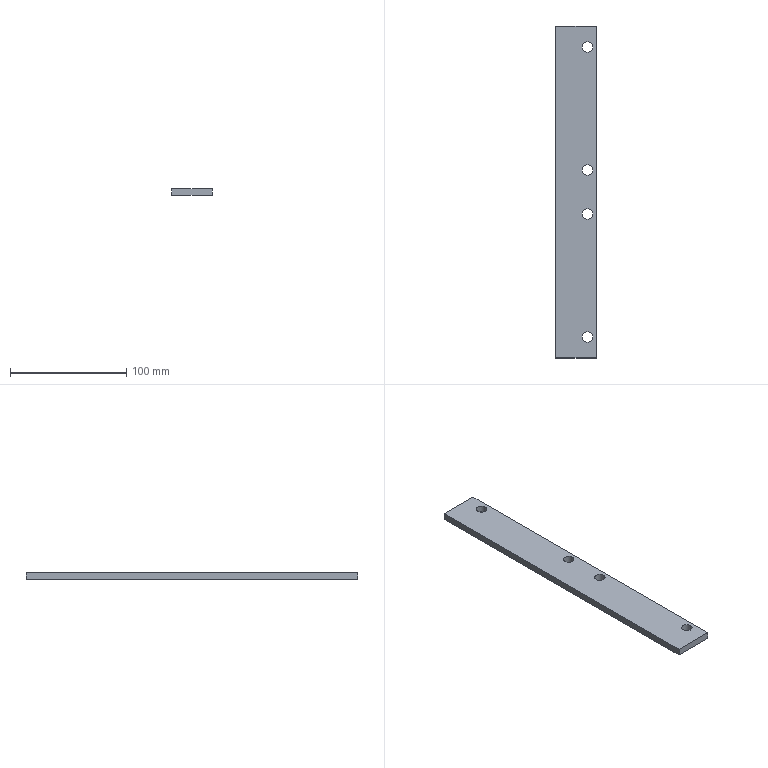Component | NX | FIXED_PLATE_8 | 1 solid | 10 faces | box 35 x 286 x 6 mm | volume 58533 mm3 | plane 6 | cylinder 4 | commonest cylinder face diameters 9 x4
STEP:
#1=CARTESIAN_POINT('',(0.,0.,0.));
#2=DIRECTION('',(0.,0.,1.));
#3=DIRECTION('',(1.,0.,0.));
#4=AXIS2_PLACEMENT_3D('',#1,#2,#3);
#5=CARTESIAN_POINT('',(1499.254,1431.,809.574));
#6=VERTEX_POINT('',#5);
#7=CARTESIAN_POINT('',(1499.254,1145.,809.574));
#8=VERTEX_POINT('',#7);
#9=CARTESIAN_POINT('',(1499.254,1431.,809.574));
#10=DIRECTION('',(-0.,-1.,0.));
#11=VECTOR('',#10,1.);
#12=LINE('',#9,#11);
#13=CARTESIAN_POINT('',(1499.254,1431.,803.574));
#14=DIRECTION('',(-1.,0.,0.));
#15=DIRECTION('',(-0.,-1.,0.));
#16=AXIS2_PLACEMENT_3D('',#13,#14,#15);
#17=PLANE('',#16);
#18=CARTESIAN_POINT('',(0.,6.));
#19=DIRECTION('',(1.,0.));
#20=VECTOR('',#19,1.);
#21=LINE('',#18,#20);
#22=(GEOMETRIC_REPRESENTATION_CONTEXT(2)PARAMETRIC_REPRESENTATION_CONTEXT()REPRESENTATION_CONTEXT('',''));
#23=DEFINITIONAL_REPRESENTATION('',(#21),#22);
#24=PCURVE('',#17,#23);
#25=CARTESIAN_POINT('',(1526.754,1163.,809.574));
#26=DIRECTION('',(0.,0.,1.));
#27=DIRECTION('',(1.,0.,0.));
#28=AXIS2_PLACEMENT_3D('',#25,#26,#27);
#29=PLANE('',#28);
#30=CARTESIAN_POINT('',(-27.5,268.));
#31=DIRECTION('',(-0.,-1.));
#32=VECTOR('',#31,1.);
#33=LINE('',#30,#32);
#34=(GEOMETRIC_REPRESENTATION_CONTEXT(2)PARAMETRIC_REPRESENTATION_CONTEXT()REPRESENTATION_CONTEXT('',''));
#35=DEFINITIONAL_REPRESENTATION('',(#33),#34);
#36=PCURVE('',#29,#35);
#37=SURFACE_CURVE('',#12,(#24,#36),.PCURVE_S1.);
#38=EDGE_CURVE('',#6,#8,#37,.T.);
#39=ORIENTED_EDGE('',*,*,#38,.F.);
#40=CARTESIAN_POINT('',(1499.254,1431.,803.574));
#41=VERTEX_POINT('',#40);
#42=CARTESIAN_POINT('',(1499.254,1431.,803.574));
#43=DIRECTION('',(0.,0.,1.));
#44=VECTOR('',#43,1.);
#45=LINE('',#42,#44);
#46=CARTESIAN_POINT('',(0.,0.));
#47=DIRECTION('',(0.,1.));
#48=VECTOR('',#47,1.);
#49=LINE('',#46,#48);
#50=(GEOMETRIC_REPRESENTATION_CONTEXT(2)PARAMETRIC_REPRESENTATION_CONTEXT()REPRESENTATION_CONTEXT('',''));
#51=DEFINITIONAL_REPRESENTATION('',(#49),#50);
#52=PCURVE('',#17,#51);
#53=CARTESIAN_POINT('',(1534.254,1431.,803.574));
#54=DIRECTION('',(0.,1.,0.));
#55=DIRECTION('',(0.,0.,1.));
#56=AXIS2_PLACEMENT_3D('',#53,#54,#55);
#57=PLANE('',#56);
#58=CARTESIAN_POINT('',(0.,-35.));
#59=DIRECTION('',(1.,0.));
#60=VECTOR('',#59,1.);
#61=LINE('',#58,#60);
#62=(GEOMETRIC_REPRESENTATION_CONTEXT(2)PARAMETRIC_REPRESENTATION_CONTEXT()REPRESENTATION_CONTEXT('',''));
#63=DEFINITIONAL_REPRESENTATION('',(#61),#62);
#64=PCURVE('',#57,#63);
#65=SURFACE_CURVE('',#45,(#52,#64),.PCURVE_S1.);
#66=EDGE_CURVE('',#41,#6,#65,.T.);
#67=ORIENTED_EDGE('',*,*,#66,.F.);
#68=CARTESIAN_POINT('',(1499.254,1145.,803.574));
#69=VERTEX_POINT('',#68);
#70=CARTESIAN_POINT('',(1499.254,1431.,803.574));
#71=DIRECTION('',(-0.,-1.,0.));
#72=VECTOR('',#71,1.);
#73=LINE('',#70,#72);
#74=CARTESIAN_POINT('',(0.,0.));
#75=DIRECTION('',(1.,0.));
#76=VECTOR('',#75,1.);
#77=LINE('',#74,#76);
#78=(GEOMETRIC_REPRESENTATION_CONTEXT(2)PARAMETRIC_REPRESENTATION_CONTEXT()REPRESENTATION_CONTEXT('',''));
#79=DEFINITIONAL_REPRESENTATION('',(#77),#78);
#80=PCURVE('',#17,#79);
#81=CARTESIAN_POINT('',(1526.754,1163.,803.574));
#82=DIRECTION('',(0.,0.,1.));
#83=DIRECTION('',(1.,0.,0.));
#84=AXIS2_PLACEMENT_3D('',#81,#82,#83);
#85=PLANE('',#84);
#86=CARTESIAN_POINT('',(-27.5,268.));
#87=DIRECTION('',(-0.,-1.));
#88=VECTOR('',#87,1.);
#89=LINE('',#86,#88);
#90=(GEOMETRIC_REPRESENTATION_CONTEXT(2)PARAMETRIC_REPRESENTATION_CONTEXT()REPRESENTATION_CONTEXT('',''));
#91=DEFINITIONAL_REPRESENTATION('',(#89),#90);
#92=PCURVE('',#85,#91);
#93=SURFACE_CURVE('',#73,(#80,#92),.PCURVE_S1.);
#94=EDGE_CURVE('',#41,#69,#93,.T.);
#95=ORIENTED_EDGE('',*,*,#94,.T.);
#96=CARTESIAN_POINT('',(1499.254,1145.,803.574));
#97=DIRECTION('',(0.,0.,1.));
#98=VECTOR('',#97,1.);
#99=LINE('',#96,#98);
#100=CARTESIAN_POINT('',(286.,0.));
#101=DIRECTION('',(0.,1.));
#102=VECTOR('',#101,1.);
#103=LINE('',#100,#102);
#104=(GEOMETRIC_REPRESENTATION_CONTEXT(2)PARAMETRIC_REPRESENTATION_CONTEXT()REPRESENTATION_CONTEXT('',''));
#105=DEFINITIONAL_REPRESENTATION('',(#103),#104);
#106=PCURVE('',#17,#105);
#107=CARTESIAN_POINT('',(1499.254,1145.,803.574));
#108=DIRECTION('',(0.,-1.,0.));
#109=DIRECTION('',(0.,0.,-1.));
#110=AXIS2_PLACEMENT_3D('',#107,#108,#109);
#111=PLANE('',#110);
#112=CARTESIAN_POINT('',(0.,0.));
#113=DIRECTION('',(-1.,0.));
#114=VECTOR('',#113,1.);
#115=LINE('',#112,#114);
#116=(GEOMETRIC_REPRESENTATION_CONTEXT(2)PARAMETRIC_REPRESENTATION_CONTEXT()REPRESENTATION_CONTEXT('',''));
#117=DEFINITIONAL_REPRESENTATION('',(#115),#116);
#118=PCURVE('',#111,#117);
#119=SURFACE_CURVE('',#99,(#106,#118),.PCURVE_S1.);
#120=EDGE_CURVE('',#69,#8,#119,.T.);
#121=ORIENTED_EDGE('',*,*,#120,.T.);
#122=EDGE_LOOP('',(#39,#67,#95,#121));
#123=FACE_BOUND('',#122,.T.);
#124=ADVANCED_FACE('',(#123),#17,.T.);
#125=CARTESIAN_POINT('',(1534.254,1145.,809.574));
#126=VERTEX_POINT('',#125);
#127=CARTESIAN_POINT('',(1499.254,1145.,809.574));
#128=DIRECTION('',(1.,0.,0.));
#129=VECTOR('',#128,1.);
#130=LINE('',#127,#129);
#131=CARTESIAN_POINT('',(-6.,0.));
#132=DIRECTION('',(0.,1.));
#133=VECTOR('',#132,1.);
#134=LINE('',#131,#133);
#135=(GEOMETRIC_REPRESENTATION_CONTEXT(2)PARAMETRIC_REPRESENTATION_CONTEXT()REPRESENTATION_CONTEXT('',''));
#136=DEFINITIONAL_REPRESENTATION('',(#134),#135);
#137=PCURVE('',#111,#136);
#138=CARTESIAN_POINT('',(-27.5,-18.));
#139=DIRECTION('',(1.,0.));
#140=VECTOR('',#139,1.);
#141=LINE('',#138,#140);
#142=(GEOMETRIC_REPRESENTATION_CONTEXT(2)PARAMETRIC_REPRESENTATION_CONTEXT()REPRESENTATION_CONTEXT('',''));
#143=DEFINITIONAL_REPRESENTATION('',(#141),#142);
#144=PCURVE('',#29,#143);
#145=SURFACE_CURVE('',#130,(#137,#144),.PCURVE_S1.);
#146=EDGE_CURVE('',#8,#126,#145,.T.);
#147=ORIENTED_EDGE('',*,*,#146,.F.);
#148=ORIENTED_EDGE('',*,*,#120,.F.);
#149=CARTESIAN_POINT('',(1534.254,1145.,803.574));
#150=VERTEX_POINT('',#149);
#151=CARTESIAN_POINT('',(1499.254,1145.,803.574));
#152=DIRECTION('',(1.,0.,0.));
#153=VECTOR('',#152,1.);
#154=LINE('',#151,#153);
#155=CARTESIAN_POINT('',(0.,0.));
#156=DIRECTION('',(0.,1.));
#157=VECTOR('',#156,1.);
#158=LINE('',#155,#157);
#159=(GEOMETRIC_REPRESENTATION_CONTEXT(2)PARAMETRIC_REPRESENTATION_CONTEXT()REPRESENTATION_CONTEXT('',''));
#160=DEFINITIONAL_REPRESENTATION('',(#158),#159);
#161=PCURVE('',#111,#160);
#162=CARTESIAN_POINT('',(-27.5,-18.));
#163=DIRECTION('',(1.,0.));
#164=VECTOR('',#163,1.);
#165=LINE('',#162,#164);
#166=(GEOMETRIC_REPRESENTATION_CONTEXT(2)PARAMETRIC_REPRESENTATION_CONTEXT()REPRESENTATION_CONTEXT('',''));
#167=DEFINITIONAL_REPRESENTATION('',(#165),#166);
#168=PCURVE('',#85,#167);
#169=SURFACE_CURVE('',#154,(#161,#168),.PCURVE_S1.);
#170=EDGE_CURVE('',#69,#150,#169,.T.);
#171=ORIENTED_EDGE('',*,*,#170,.T.);
#172=CARTESIAN_POINT('',(1534.254,1145.,803.574));
#173=DIRECTION('',(0.,0.,1.));
#174=VECTOR('',#173,1.);
#175=LINE('',#172,#174);
#176=CARTESIAN_POINT('',(0.,35.));
#177=DIRECTION('',(-1.,0.));
#178=VECTOR('',#177,1.);
#179=LINE('',#176,#178);
#180=(GEOMETRIC_REPRESENTATION_CONTEXT(2)PARAMETRIC_REPRESENTATION_CONTEXT()REPRESENTATION_CONTEXT('',''));
#181=DEFINITIONAL_REPRESENTATION('',(#179),#180);
#182=PCURVE('',#111,#181);
#183=CARTESIAN_POINT('',(1534.254,1145.,803.574));
#184=DIRECTION('',(1.,-0.,0.));
#185=DIRECTION('',(0.,1.,0.));
#186=AXIS2_PLACEMENT_3D('',#183,#184,#185);
#187=PLANE('',#186);
#188=CARTESIAN_POINT('',(0.,0.));
#189=DIRECTION('',(0.,1.));
#190=VECTOR('',#189,1.);
#191=LINE('',#188,#190);
#192=(GEOMETRIC_REPRESENTATION_CONTEXT(2)PARAMETRIC_REPRESENTATION_CONTEXT()REPRESENTATION_CONTEXT('',''));
#193=DEFINITIONAL_REPRESENTATION('',(#191),#192);
#194=PCURVE('',#187,#193);
#195=SURFACE_CURVE('',#175,(#182,#194),.PCURVE_S1.);
#196=EDGE_CURVE('',#150,#126,#195,.T.);
#197=ORIENTED_EDGE('',*,*,#196,.T.);
#198=EDGE_LOOP('',(#147,#148,#171,#197));
#199=FACE_BOUND('',#198,.T.);
#200=ADVANCED_FACE('',(#199),#111,.T.);
#201=CARTESIAN_POINT('',(1534.254,1431.,809.574));
#202=VERTEX_POINT('',#201);
#203=CARTESIAN_POINT('',(1534.254,1145.,809.574));
#204=DIRECTION('',(0.,1.,0.));
#205=VECTOR('',#204,1.);
#206=LINE('',#203,#205);
#207=CARTESIAN_POINT('',(0.,6.));
#208=DIRECTION('',(1.,0.));
#209=VECTOR('',#208,1.);
#210=LINE('',#207,#209);
#211=(GEOMETRIC_REPRESENTATION_CONTEXT(2)PARAMETRIC_REPRESENTATION_CONTEXT()REPRESENTATION_CONTEXT('',''));
#212=DEFINITIONAL_REPRESENTATION('',(#210),#211);
#213=PCURVE('',#187,#212);
#214=CARTESIAN_POINT('',(7.5,-18.));
#215=DIRECTION('',(0.,1.));
#216=VECTOR('',#215,1.);
#217=LINE('',#214,#216);
#218=(GEOMETRIC_REPRESENTATION_CONTEXT(2)PARAMETRIC_REPRESENTATION_CONTEXT()REPRESENTATION_CONTEXT('',''));
#219=DEFINITIONAL_REPRESENTATION('',(#217),#218);
#220=PCURVE('',#29,#219);
#221=SURFACE_CURVE('',#206,(#213,#220),.PCURVE_S1.);
#222=EDGE_CURVE('',#126,#202,#221,.T.);
#223=ORIENTED_EDGE('',*,*,#222,.F.);
#224=ORIENTED_EDGE('',*,*,#196,.F.);
#225=CARTESIAN_POINT('',(1534.254,1431.,803.574));
#226=VERTEX_POINT('',#225);
#227=CARTESIAN_POINT('',(1534.254,1145.,803.574));
#228=DIRECTION('',(0.,1.,0.));
#229=VECTOR('',#228,1.);
#230=LINE('',#227,#229);
#231=CARTESIAN_POINT('',(0.,0.));
#232=DIRECTION('',(1.,0.));
#233=VECTOR('',#232,1.);
#234=LINE('',#231,#233);
#235=(GEOMETRIC_REPRESENTATION_CONTEXT(2)PARAMETRIC_REPRESENTATION_CONTEXT()REPRESENTATION_CONTEXT('',''));
#236=DEFINITIONAL_REPRESENTATION('',(#234),#235);
#237=PCURVE('',#187,#236);
#238=CARTESIAN_POINT('',(7.5,-18.));
#239=DIRECTION('',(0.,1.));
#240=VECTOR('',#239,1.);
#241=LINE('',#238,#240);
#242=(GEOMETRIC_REPRESENTATION_CONTEXT(2)PARAMETRIC_REPRESENTATION_CONTEXT()REPRESENTATION_CONTEXT('',''));
#243=DEFINITIONAL_REPRESENTATION('',(#241),#242);
#244=PCURVE('',#85,#243);
#245=SURFACE_CURVE('',#230,(#237,#244),.PCURVE_S1.);
#246=EDGE_CURVE('',#150,#226,#245,.T.);
#247=ORIENTED_EDGE('',*,*,#246,.T.);
#248=CARTESIAN_POINT('',(1534.254,1431.,803.574));
#249=DIRECTION('',(0.,0.,1.));
#250=VECTOR('',#249,1.);
#251=LINE('',#248,#250);
#252=CARTESIAN_POINT('',(286.,0.));
#253=DIRECTION('',(0.,1.));
#254=VECTOR('',#253,1.);
#255=LINE('',#252,#254);
#256=(GEOMETRIC_REPRESENTATION_CONTEXT(2)PARAMETRIC_REPRESENTATION_CONTEXT()REPRESENTATION_CONTEXT('',''));
#257=DEFINITIONAL_REPRESENTATION('',(#255),#256);
#258=PCURVE('',#187,#257);
#259=CARTESIAN_POINT('',(0.,0.));
#260=DIRECTION('',(1.,0.));
#261=VECTOR('',#260,1.);
#262=LINE('',#259,#261);
#263=(GEOMETRIC_REPRESENTATION_CONTEXT(2)PARAMETRIC_REPRESENTATION_CONTEXT()REPRESENTATION_CONTEXT('',''));
#264=DEFINITIONAL_REPRESENTATION('',(#262),#263);
#265=PCURVE('',#57,#264);
#266=SURFACE_CURVE('',#251,(#258,#265),.PCURVE_S1.);
#267=EDGE_CURVE('',#226,#202,#266,.T.);
#268=ORIENTED_EDGE('',*,*,#267,.T.);
#269=EDGE_LOOP('',(#223,#224,#247,#268));
#270=FACE_BOUND('',#269,.T.);
#271=ADVANCED_FACE('',(#270),#187,.T.);
#272=CARTESIAN_POINT('',(1531.254,1307.,803.574));
#273=VERTEX_POINT('',#272);
#274=CARTESIAN_POINT('',(1526.754,1307.,803.574));
#275=DIRECTION('',(0.,0.,1.));
#276=DIRECTION('',(1.,0.,0.));
#277=AXIS2_PLACEMENT_3D('',#274,#275,#276);
#278=CIRCLE('',#277,4.5);
#279=CARTESIAN_POINT('',(1526.754,1307.,803.574));
#280=DIRECTION('',(0.,0.,1.));
#281=DIRECTION('',(1.,0.,0.));
#282=AXIS2_PLACEMENT_3D('',#279,#280,#281);
#283=CYLINDRICAL_SURFACE('',#282,4.5);
#284=CARTESIAN_POINT('',(0.,0.));
#285=DIRECTION('',(1.,0.));
#286=VECTOR('',#285,1.);
#287=LINE('',#284,#286);
#288=(GEOMETRIC_REPRESENTATION_CONTEXT(2)PARAMETRIC_REPRESENTATION_CONTEXT()REPRESENTATION_CONTEXT('',''));
#289=DEFINITIONAL_REPRESENTATION('',(#287),#288);
#290=PCURVE('',#283,#289);
#291=CARTESIAN_POINT('',(0.,144.));
#292=DIRECTION('',(1.,0.));
#293=AXIS2_PLACEMENT_2D('',#291,#292);
#294=CIRCLE('',#293,4.5);
#295=(GEOMETRIC_REPRESENTATION_CONTEXT(2)PARAMETRIC_REPRESENTATION_CONTEXT()REPRESENTATION_CONTEXT('',''));
#296=DEFINITIONAL_REPRESENTATION('',(#294),#295);
#297=PCURVE('',#85,#296);
#298=SURFACE_CURVE('',#278,(#290,#297),.PCURVE_S1.);
#299=EDGE_CURVE('',#273,#273,#298,.T.);
#300=ORIENTED_EDGE('',*,*,#299,.T.);
#301=CARTESIAN_POINT('',(1531.254,1307.,809.574));
#302=VERTEX_POINT('',#301);
#303=CARTESIAN_POINT('',(1531.254,1307.,803.574));
#304=CARTESIAN_POINT('',(1531.254,1307.,809.574));
#305=B_SPLINE_CURVE_WITH_KNOTS('',1,(#303,#304),.UNSPECIFIED.,.F.,.F.,(2,2),(0.,6.),.PIECEWISE_BEZIER_KNOTS.);
#306=CARTESIAN_POINT('',(6.283,0.));
#307=DIRECTION('',(0.,1.));
#308=VECTOR('',#307,1.);
#309=LINE('',#306,#308);
#310=(GEOMETRIC_REPRESENTATION_CONTEXT(2)PARAMETRIC_REPRESENTATION_CONTEXT()REPRESENTATION_CONTEXT('',''));
#311=DEFINITIONAL_REPRESENTATION('',(#309),#310);
#312=PCURVE('',#283,#311);
#313=CARTESIAN_POINT('',(0.,0.));
#314=DIRECTION('',(0.,1.));
#315=VECTOR('',#314,1.);
#316=LINE('',#313,#315);
#317=(GEOMETRIC_REPRESENTATION_CONTEXT(2)PARAMETRIC_REPRESENTATION_CONTEXT()REPRESENTATION_CONTEXT('',''));
#318=DEFINITIONAL_REPRESENTATION('',(#316),#317);
#319=PCURVE('',#283,#318);
#320=SEAM_CURVE('',#305,(#312,#319),.PCURVE_S1.);
#321=EDGE_CURVE('',#273,#302,#320,.T.);
#322=ORIENTED_EDGE('',*,*,#321,.T.);
#323=CARTESIAN_POINT('',(1526.754,1307.,809.574));
#324=DIRECTION('',(0.,0.,1.));
#325=DIRECTION('',(1.,0.,0.));
#326=AXIS2_PLACEMENT_3D('',#323,#324,#325);
#327=CIRCLE('',#326,4.5);
#328=CARTESIAN_POINT('',(0.,6.));
#329=DIRECTION('',(1.,0.));
#330=VECTOR('',#329,1.);
#331=LINE('',#328,#330);
#332=(GEOMETRIC_REPRESENTATION_CONTEXT(2)PARAMETRIC_REPRESENTATION_CONTEXT()REPRESENTATION_CONTEXT('',''));
#333=DEFINITIONAL_REPRESENTATION('',(#331),#332);
#334=PCURVE('',#283,#333);
#335=CARTESIAN_POINT('',(0.,144.));
#336=DIRECTION('',(1.,0.));
#337=AXIS2_PLACEMENT_2D('',#335,#336);
#338=CIRCLE('',#337,4.5);
#339=(GEOMETRIC_REPRESENTATION_CONTEXT(2)PARAMETRIC_REPRESENTATION_CONTEXT()REPRESENTATION_CONTEXT('',''));
#340=DEFINITIONAL_REPRESENTATION('',(#338),#339);
#341=PCURVE('',#29,#340);
#342=SURFACE_CURVE('',#327,(#334,#341),.PCURVE_S1.);
#343=EDGE_CURVE('',#302,#302,#342,.T.);
#344=ORIENTED_EDGE('',*,*,#343,.F.);
#345=ORIENTED_EDGE('',*,*,#321,.F.);
#346=EDGE_LOOP('',(#300,#322,#344,#345));
#347=FACE_BOUND('',#346,.F.);
#348=ADVANCED_FACE('',(#347),#283,.F.);
#349=CARTESIAN_POINT('',(1531.254,1269.,803.574));
#350=VERTEX_POINT('',#349);
#351=CARTESIAN_POINT('',(1526.754,1269.,803.574));
#352=DIRECTION('',(0.,0.,1.));
#353=DIRECTION('',(1.,0.,0.));
#354=AXIS2_PLACEMENT_3D('',#351,#352,#353);
#355=CIRCLE('',#354,4.5);
#356=CARTESIAN_POINT('',(1526.754,1269.,803.574));
#357=DIRECTION('',(0.,0.,1.));
#358=DIRECTION('',(1.,0.,0.));
#359=AXIS2_PLACEMENT_3D('',#356,#357,#358);
#360=CYLINDRICAL_SURFACE('',#359,4.5);
#361=CARTESIAN_POINT('',(0.,0.));
#362=DIRECTION('',(1.,0.));
#363=VECTOR('',#362,1.);
#364=LINE('',#361,#363);
#365=(GEOMETRIC_REPRESENTATION_CONTEXT(2)PARAMETRIC_REPRESENTATION_CONTEXT()REPRESENTATION_CONTEXT('',''));
#366=DEFINITIONAL_REPRESENTATION('',(#364),#365);
#367=PCURVE('',#360,#366);
#368=CARTESIAN_POINT('',(0.,106.));
#369=DIRECTION('',(1.,0.));
#370=AXIS2_PLACEMENT_2D('',#368,#369);
#371=CIRCLE('',#370,4.5);
#372=(GEOMETRIC_REPRESENTATION_CONTEXT(2)PARAMETRIC_REPRESENTATION_CONTEXT()REPRESENTATION_CONTEXT('',''));
#373=DEFINITIONAL_REPRESENTATION('',(#371),#372);
#374=PCURVE('',#85,#373);
#375=SURFACE_CURVE('',#355,(#367,#374),.PCURVE_S1.);
#376=EDGE_CURVE('',#350,#350,#375,.T.);
#377=ORIENTED_EDGE('',*,*,#376,.T.);
#378=CARTESIAN_POINT('',(1531.254,1269.,809.574));
#379=VERTEX_POINT('',#378);
#380=CARTESIAN_POINT('',(1531.254,1269.,803.574));
#381=CARTESIAN_POINT('',(1531.254,1269.,809.574));
#382=B_SPLINE_CURVE_WITH_KNOTS('',1,(#380,#381),.UNSPECIFIED.,.F.,.F.,(2,2),(0.,6.),.PIECEWISE_BEZIER_KNOTS.);
#383=CARTESIAN_POINT('',(6.283,0.));
#384=DIRECTION('',(0.,1.));
#385=VECTOR('',#384,1.);
#386=LINE('',#383,#385);
#387=(GEOMETRIC_REPRESENTATION_CONTEXT(2)PARAMETRIC_REPRESENTATION_CONTEXT()REPRESENTATION_CONTEXT('',''));
#388=DEFINITIONAL_REPRESENTATION('',(#386),#387);
#389=PCURVE('',#360,#388);
#390=CARTESIAN_POINT('',(0.,0.));
#391=DIRECTION('',(0.,1.));
#392=VECTOR('',#391,1.);
#393=LINE('',#390,#392);
#394=(GEOMETRIC_REPRESENTATION_CONTEXT(2)PARAMETRIC_REPRESENTATION_CONTEXT()REPRESENTATION_CONTEXT('',''));
#395=DEFINITIONAL_REPRESENTATION('',(#393),#394);
#396=PCURVE('',#360,#395);
#397=SEAM_CURVE('',#382,(#389,#396),.PCURVE_S1.);
#398=EDGE_CURVE('',#350,#379,#397,.T.);
#399=ORIENTED_EDGE('',*,*,#398,.T.);
#400=CARTESIAN_POINT('',(1526.754,1269.,809.574));
#401=DIRECTION('',(0.,0.,1.));
#402=DIRECTION('',(1.,0.,0.));
#403=AXIS2_PLACEMENT_3D('',#400,#401,#402);
#404=CIRCLE('',#403,4.5);
#405=CARTESIAN_POINT('',(0.,6.));
#406=DIRECTION('',(1.,0.));
#407=VECTOR('',#406,1.);
#408=LINE('',#405,#407);
#409=(GEOMETRIC_REPRESENTATION_CONTEXT(2)PARAMETRIC_REPRESENTATION_CONTEXT()REPRESENTATION_CONTEXT('',''));
#410=DEFINITIONAL_REPRESENTATION('',(#408),#409);
#411=PCURVE('',#360,#410);
#412=CARTESIAN_POINT('',(0.,106.));
#413=DIRECTION('',(1.,0.));
#414=AXIS2_PLACEMENT_2D('',#412,#413);
#415=CIRCLE('',#414,4.5);
#416=(GEOMETRIC_REPRESENTATION_CONTEXT(2)PARAMETRIC_REPRESENTATION_CONTEXT()REPRESENTATION_CONTEXT('',''));
#417=DEFINITIONAL_REPRESENTATION('',(#415),#416);
#418=PCURVE('',#29,#417);
#419=SURFACE_CURVE('',#404,(#411,#418),.PCURVE_S1.);
#420=EDGE_CURVE('',#379,#379,#419,.T.);
#421=ORIENTED_EDGE('',*,*,#420,.F.);
#422=ORIENTED_EDGE('',*,*,#398,.F.);
#423=EDGE_LOOP('',(#377,#399,#421,#422));
#424=FACE_BOUND('',#423,.F.);
#425=ADVANCED_FACE('',(#424),#360,.F.);
#426=CARTESIAN_POINT('',(1531.254,1163.,803.574));
#427=VERTEX_POINT('',#426);
#428=CARTESIAN_POINT('',(1526.754,1163.,803.574));
#429=DIRECTION('',(0.,0.,1.));
#430=DIRECTION('',(1.,0.,0.));
#431=AXIS2_PLACEMENT_3D('',#428,#429,#430);
#432=CIRCLE('',#431,4.5);
#433=CARTESIAN_POINT('',(1526.754,1163.,803.574));
#434=DIRECTION('',(0.,0.,1.));
#435=DIRECTION('',(1.,0.,0.));
#436=AXIS2_PLACEMENT_3D('',#433,#434,#435);
#437=CYLINDRICAL_SURFACE('',#436,4.5);
#438=CARTESIAN_POINT('',(0.,0.));
#439=DIRECTION('',(1.,0.));
#440=VECTOR('',#439,1.);
#441=LINE('',#438,#440);
#442=(GEOMETRIC_REPRESENTATION_CONTEXT(2)PARAMETRIC_REPRESENTATION_CONTEXT()REPRESENTATION_CONTEXT('',''));
#443=DEFINITIONAL_REPRESENTATION('',(#441),#442);
#444=PCURVE('',#437,#443);
#445=CARTESIAN_POINT('',(0.,0.));
#446=DIRECTION('',(1.,0.));
#447=AXIS2_PLACEMENT_2D('',#445,#446);
#448=CIRCLE('',#447,4.5);
#449=(GEOMETRIC_REPRESENTATION_CONTEXT(2)PARAMETRIC_REPRESENTATION_CONTEXT()REPRESENTATION_CONTEXT('',''));
#450=DEFINITIONAL_REPRESENTATION('',(#448),#449);
#451=PCURVE('',#85,#450);
#452=SURFACE_CURVE('',#432,(#444,#451),.PCURVE_S1.);
#453=EDGE_CURVE('',#427,#427,#452,.T.);
#454=ORIENTED_EDGE('',*,*,#453,.T.);
#455=CARTESIAN_POINT('',(1531.254,1163.,809.574));
#456=VERTEX_POINT('',#455);
#457=CARTESIAN_POINT('',(1531.254,1163.,803.574));
#458=CARTESIAN_POINT('',(1531.254,1163.,809.574));
#459=B_SPLINE_CURVE_WITH_KNOTS('',1,(#457,#458),.UNSPECIFIED.,.F.,.F.,(2,2),(0.,6.),.PIECEWISE_BEZIER_KNOTS.);
#460=CARTESIAN_POINT('',(6.283,0.));
#461=DIRECTION('',(0.,1.));
#462=VECTOR('',#461,1.);
#463=LINE('',#460,#462);
#464=(GEOMETRIC_REPRESENTATION_CONTEXT(2)PARAMETRIC_REPRESENTATION_CONTEXT()REPRESENTATION_CONTEXT('',''));
#465=DEFINITIONAL_REPRESENTATION('',(#463),#464);
#466=PCURVE('',#437,#465);
#467=CARTESIAN_POINT('',(0.,0.));
#468=DIRECTION('',(0.,1.));
#469=VECTOR('',#468,1.);
#470=LINE('',#467,#469);
#471=(GEOMETRIC_REPRESENTATION_CONTEXT(2)PARAMETRIC_REPRESENTATION_CONTEXT()REPRESENTATION_CONTEXT('',''));
#472=DEFINITIONAL_REPRESENTATION('',(#470),#471);
#473=PCURVE('',#437,#472);
#474=SEAM_CURVE('',#459,(#466,#473),.PCURVE_S1.);
#475=EDGE_CURVE('',#427,#456,#474,.T.);
#476=ORIENTED_EDGE('',*,*,#475,.T.);
#477=CARTESIAN_POINT('',(1526.754,1163.,809.574));
#478=DIRECTION('',(0.,0.,1.));
#479=DIRECTION('',(1.,0.,0.));
#480=AXIS2_PLACEMENT_3D('',#477,#478,#479);
#481=CIRCLE('',#480,4.5);
#482=CARTESIAN_POINT('',(0.,6.));
#483=DIRECTION('',(1.,0.));
#484=VECTOR('',#483,1.);
#485=LINE('',#482,#484);
#486=(GEOMETRIC_REPRESENTATION_CONTEXT(2)PARAMETRIC_REPRESENTATION_CONTEXT()REPRESENTATION_CONTEXT('',''));
#487=DEFINITIONAL_REPRESENTATION('',(#485),#486);
#488=PCURVE('',#437,#487);
#489=CARTESIAN_POINT('',(0.,0.));
#490=DIRECTION('',(1.,0.));
#491=AXIS2_PLACEMENT_2D('',#489,#490);
#492=CIRCLE('',#491,4.5);
#493=(GEOMETRIC_REPRESENTATION_CONTEXT(2)PARAMETRIC_REPRESENTATION_CONTEXT()REPRESENTATION_CONTEXT('',''));
#494=DEFINITIONAL_REPRESENTATION('',(#492),#493);
#495=PCURVE('',#29,#494);
#496=SURFACE_CURVE('',#481,(#488,#495),.PCURVE_S1.);
#497=EDGE_CURVE('',#456,#456,#496,.T.);
#498=ORIENTED_EDGE('',*,*,#497,.F.);
#499=ORIENTED_EDGE('',*,*,#475,.F.);
#500=EDGE_LOOP('',(#454,#476,#498,#499));
#501=FACE_BOUND('',#500,.F.);
#502=ADVANCED_FACE('',(#501),#437,.F.);
#503=CARTESIAN_POINT('',(1534.254,1431.,809.574));
#504=DIRECTION('',(-1.,0.,0.));
#505=VECTOR('',#504,1.);
#506=LINE('',#503,#505);
#507=CARTESIAN_POINT('',(6.,0.));
#508=DIRECTION('',(0.,-1.));
#509=VECTOR('',#508,1.);
#510=LINE('',#507,#509);
#511=(GEOMETRIC_REPRESENTATION_CONTEXT(2)PARAMETRIC_REPRESENTATION_CONTEXT()REPRESENTATION_CONTEXT('',''));
#512=DEFINITIONAL_REPRESENTATION('',(#510),#511);
#513=PCURVE('',#57,#512);
#514=CARTESIAN_POINT('',(7.5,268.));
#515=DIRECTION('',(-1.,0.));
#516=VECTOR('',#515,1.);
#517=LINE('',#514,#516);
#518=(GEOMETRIC_REPRESENTATION_CONTEXT(2)PARAMETRIC_REPRESENTATION_CONTEXT()REPRESENTATION_CONTEXT('',''));
#519=DEFINITIONAL_REPRESENTATION('',(#517),#518);
#520=PCURVE('',#29,#519);
#521=SURFACE_CURVE('',#506,(#513,#520),.PCURVE_S1.);
#522=EDGE_CURVE('',#202,#6,#521,.T.);
#523=ORIENTED_EDGE('',*,*,#522,.F.);
#524=ORIENTED_EDGE('',*,*,#267,.F.);
#525=CARTESIAN_POINT('',(1534.254,1431.,803.574));
#526=DIRECTION('',(-1.,0.,0.));
#527=VECTOR('',#526,1.);
#528=LINE('',#525,#527);
#529=CARTESIAN_POINT('',(0.,0.));
#530=DIRECTION('',(0.,-1.));
#531=VECTOR('',#530,1.);
#532=LINE('',#529,#531);
#533=(GEOMETRIC_REPRESENTATION_CONTEXT(2)PARAMETRIC_REPRESENTATION_CONTEXT()REPRESENTATION_CONTEXT('',''));
#534=DEFINITIONAL_REPRESENTATION('',(#532),#533);
#535=PCURVE('',#57,#534);
#536=CARTESIAN_POINT('',(7.5,268.));
#537=DIRECTION('',(-1.,0.));
#538=VECTOR('',#537,1.);
#539=LINE('',#536,#538);
#540=(GEOMETRIC_REPRESENTATION_CONTEXT(2)PARAMETRIC_REPRESENTATION_CONTEXT()REPRESENTATION_CONTEXT('',''));
#541=DEFINITIONAL_REPRESENTATION('',(#539),#540);
#542=PCURVE('',#85,#541);
#543=SURFACE_CURVE('',#528,(#535,#542),.PCURVE_S1.);
#544=EDGE_CURVE('',#226,#41,#543,.T.);
#545=ORIENTED_EDGE('',*,*,#544,.T.);
#546=ORIENTED_EDGE('',*,*,#66,.T.);
#547=EDGE_LOOP('',(#523,#524,#545,#546));
#548=FACE_BOUND('',#547,.T.);
#549=ADVANCED_FACE('',(#548),#57,.T.);
#550=CARTESIAN_POINT('',(1531.254,1413.,803.574));
#551=VERTEX_POINT('',#550);
#552=CARTESIAN_POINT('',(1526.754,1413.,803.574));
#553=DIRECTION('',(0.,0.,1.));
#554=DIRECTION('',(1.,0.,0.));
#555=AXIS2_PLACEMENT_3D('',#552,#553,#554);
#556=CIRCLE('',#555,4.5);
#557=CARTESIAN_POINT('',(1526.754,1413.,803.574));
#558=DIRECTION('',(0.,0.,1.));
#559=DIRECTION('',(1.,0.,0.));
#560=AXIS2_PLACEMENT_3D('',#557,#558,#559);
#561=CYLINDRICAL_SURFACE('',#560,4.5);
#562=CARTESIAN_POINT('',(0.,0.));
#563=DIRECTION('',(1.,0.));
#564=VECTOR('',#563,1.);
#565=LINE('',#562,#564);
#566=(GEOMETRIC_REPRESENTATION_CONTEXT(2)PARAMETRIC_REPRESENTATION_CONTEXT()REPRESENTATION_CONTEXT('',''));
#567=DEFINITIONAL_REPRESENTATION('',(#565),#566);
#568=PCURVE('',#561,#567);
#569=CARTESIAN_POINT('',(0.,250.));
#570=DIRECTION('',(1.,0.));
#571=AXIS2_PLACEMENT_2D('',#569,#570);
#572=CIRCLE('',#571,4.5);
#573=(GEOMETRIC_REPRESENTATION_CONTEXT(2)PARAMETRIC_REPRESENTATION_CONTEXT()REPRESENTATION_CONTEXT('',''));
#574=DEFINITIONAL_REPRESENTATION('',(#572),#573);
#575=PCURVE('',#85,#574);
#576=SURFACE_CURVE('',#556,(#568,#575),.PCURVE_S1.);
#577=EDGE_CURVE('',#551,#551,#576,.T.);
#578=ORIENTED_EDGE('',*,*,#577,.T.);
#579=CARTESIAN_POINT('',(1531.254,1413.,809.574));
#580=VERTEX_POINT('',#579);
#581=CARTESIAN_POINT('',(1531.254,1413.,803.574));
#582=CARTESIAN_POINT('',(1531.254,1413.,809.574));
#583=B_SPLINE_CURVE_WITH_KNOTS('',1,(#581,#582),.UNSPECIFIED.,.F.,.F.,(2,2),(0.,6.),.PIECEWISE_BEZIER_KNOTS.);
#584=CARTESIAN_POINT('',(6.283,0.));
#585=DIRECTION('',(0.,1.));
#586=VECTOR('',#585,1.);
#587=LINE('',#584,#586);
#588=(GEOMETRIC_REPRESENTATION_CONTEXT(2)PARAMETRIC_REPRESENTATION_CONTEXT()REPRESENTATION_CONTEXT('',''));
#589=DEFINITIONAL_REPRESENTATION('',(#587),#588);
#590=PCURVE('',#561,#589);
#591=CARTESIAN_POINT('',(0.,0.));
#592=DIRECTION('',(0.,1.));
#593=VECTOR('',#592,1.);
#594=LINE('',#591,#593);
#595=(GEOMETRIC_REPRESENTATION_CONTEXT(2)PARAMETRIC_REPRESENTATION_CONTEXT()REPRESENTATION_CONTEXT('',''));
#596=DEFINITIONAL_REPRESENTATION('',(#594),#595);
#597=PCURVE('',#561,#596);
#598=SEAM_CURVE('',#583,(#590,#597),.PCURVE_S1.);
#599=EDGE_CURVE('',#551,#580,#598,.T.);
#600=ORIENTED_EDGE('',*,*,#599,.T.);
#601=CARTESIAN_POINT('',(1526.754,1413.,809.574));
#602=DIRECTION('',(0.,0.,1.));
#603=DIRECTION('',(1.,0.,0.));
#604=AXIS2_PLACEMENT_3D('',#601,#602,#603);
#605=CIRCLE('',#604,4.5);
#606=CARTESIAN_POINT('',(0.,6.));
#607=DIRECTION('',(1.,0.));
#608=VECTOR('',#607,1.);
#609=LINE('',#606,#608);
#610=(GEOMETRIC_REPRESENTATION_CONTEXT(2)PARAMETRIC_REPRESENTATION_CONTEXT()REPRESENTATION_CONTEXT('',''));
#611=DEFINITIONAL_REPRESENTATION('',(#609),#610);
#612=PCURVE('',#561,#611);
#613=CARTESIAN_POINT('',(0.,250.));
#614=DIRECTION('',(1.,0.));
#615=AXIS2_PLACEMENT_2D('',#613,#614);
#616=CIRCLE('',#615,4.5);
#617=(GEOMETRIC_REPRESENTATION_CONTEXT(2)PARAMETRIC_REPRESENTATION_CONTEXT()REPRESENTATION_CONTEXT('',''));
#618=DEFINITIONAL_REPRESENTATION('',(#616),#617);
#619=PCURVE('',#29,#618);
#620=SURFACE_CURVE('',#605,(#612,#619),.PCURVE_S1.);
#621=EDGE_CURVE('',#580,#580,#620,.T.);
#622=ORIENTED_EDGE('',*,*,#621,.F.);
#623=ORIENTED_EDGE('',*,*,#599,.F.);
#624=EDGE_LOOP('',(#578,#600,#622,#623));
#625=FACE_BOUND('',#624,.F.);
#626=ADVANCED_FACE('',(#625),#561,.F.);
#627=ORIENTED_EDGE('',*,*,#94,.F.);
#628=ORIENTED_EDGE('',*,*,#544,.F.);
#629=ORIENTED_EDGE('',*,*,#246,.F.);
#630=ORIENTED_EDGE('',*,*,#170,.F.);
#631=EDGE_LOOP('',(#627,#628,#629,#630));
#632=FACE_BOUND('',#631,.T.);
#633=ORIENTED_EDGE('',*,*,#453,.T.);
#634=EDGE_LOOP('',(#633));
#635=FACE_BOUND('',#634,.T.);
#636=ORIENTED_EDGE('',*,*,#376,.T.);
#637=EDGE_LOOP('',(#636));
#638=FACE_BOUND('',#637,.T.);
#639=ORIENTED_EDGE('',*,*,#299,.T.);
#640=EDGE_LOOP('',(#639));
#641=FACE_BOUND('',#640,.T.);
#642=ORIENTED_EDGE('',*,*,#577,.T.);
#643=EDGE_LOOP('',(#642));
#644=FACE_BOUND('',#643,.T.);
#645=ADVANCED_FACE('',(#632,#635,#638,#641,#644),#85,.F.);
#646=ORIENTED_EDGE('',*,*,#38,.T.);
#647=ORIENTED_EDGE('',*,*,#146,.T.);
#648=ORIENTED_EDGE('',*,*,#222,.T.);
#649=ORIENTED_EDGE('',*,*,#522,.T.);
#650=EDGE_LOOP('',(#646,#647,#648,#649));
#651=FACE_BOUND('',#650,.T.);
#652=ORIENTED_EDGE('',*,*,#497,.F.);
#653=EDGE_LOOP('',(#652));
#654=FACE_BOUND('',#653,.T.);
#655=ORIENTED_EDGE('',*,*,#420,.F.);
#656=EDGE_LOOP('',(#655));
#657=FACE_BOUND('',#656,.T.);
#658=ORIENTED_EDGE('',*,*,#343,.F.);
#659=EDGE_LOOP('',(#658));
#660=FACE_BOUND('',#659,.T.);
#661=ORIENTED_EDGE('',*,*,#621,.F.);
#662=EDGE_LOOP('',(#661));
#663=FACE_BOUND('',#662,.T.);
#664=ADVANCED_FACE('',(#651,#654,#657,#660,#663),#29,.T.);
#665=CLOSED_SHELL('',(#124,#200,#271,#348,#425,#502,#549,#626,#645,#664));
#666=MANIFOLD_SOLID_BREP('',#665);
#667=(LENGTH_UNIT()NAMED_UNIT(*)SI_UNIT(.MILLI.,.METRE.));
#668=UNCERTAINTY_MEASURE_WITH_UNIT(LENGTH_MEASURE(0.000005),#667,'','');
#669=(NAMED_UNIT(*)PLANE_ANGLE_UNIT()SI_UNIT($,.RADIAN.));
#670=(NAMED_UNIT(*)SI_UNIT($,.STERADIAN.)SOLID_ANGLE_UNIT());
#671=(GEOMETRIC_REPRESENTATION_CONTEXT(3)GLOBAL_UNCERTAINTY_ASSIGNED_CONTEXT((#668))GLOBAL_UNIT_ASSIGNED_CONTEXT((#667,#669,#670))REPRESENTATION_CONTEXT('',''));
#672=ADVANCED_BREP_SHAPE_REPRESENTATION('',(#4,#666),#671);